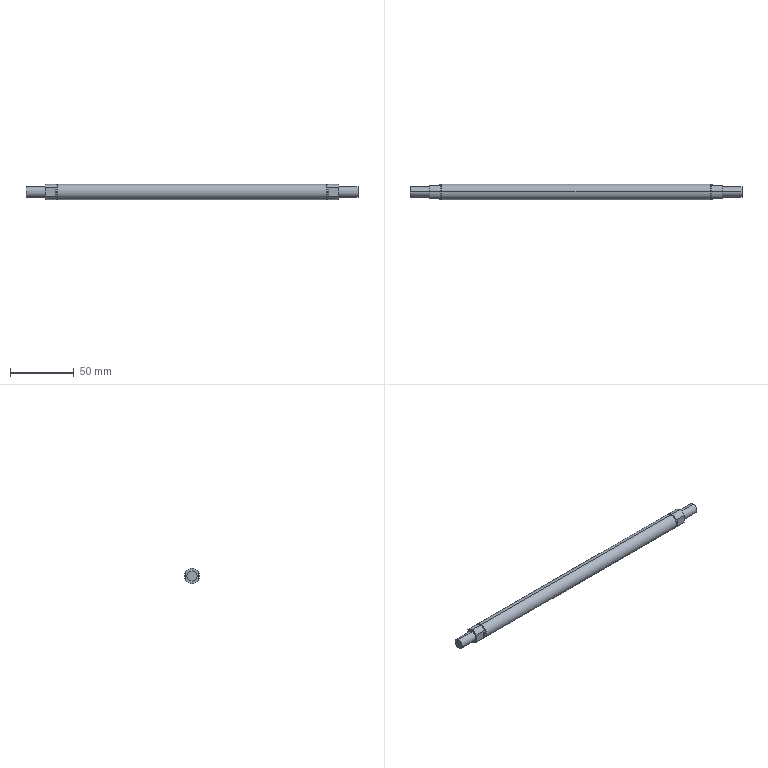Component | SolidWorks | GuideWheelAssembly3-1_RollerAxis2-1 | 1 solid | 30 faces | box 260 x 12 x 12 mm | volume 27307 mm3 | plane 16 | cylinder 14 | commonest cylinder face diameters 12 x6 10 x4 8 x4
build123d program:
from build123d import *

# Parameters (mm, degrees)
SKETCH1_R           = 6
BOSS_EXTRUDE1_DEPTH = 115
SKETCH3_R           = 4
BOSS_EXTRUDE2_DEPTH = 15
CUT_EXTRUDE7_START  = -8
CUT_EXTRUDE7_DEPTH  = 8
SKETCH20_W          = 1
SKETCH20_H          = 1


with BuildPart() as part:
    # Sketch1 → Boss-Extrude1 (new body)
    with BuildSketch(Plane(origin=(0, 0, 0), x_dir=(1, 0, 0), z_dir=(0, 1, 0))):
        with Locations(Location((0, 0, 0), (0, 0, 270))):
            Circle(SKETCH1_R)
    extrude(amount=BOSS_EXTRUDE1_DEPTH)

    # Sketch3 → Boss-Extrude2 (add)
    with BuildSketch(Plane(origin=(0, 115, 0), x_dir=(1, 0, 0), z_dir=(0, 1, 0))):
        with Locations(Location((0, 0, 0), (0, 0, 270))):
            Circle(SKETCH3_R)
    extrude(amount=BOSS_EXTRUDE2_DEPTH)

    # Sketch17 → Cut-Extrude7 (cut)
    with BuildSketch(Plane(origin=(0, 115, 0), x_dir=(1, 0, 0), z_dir=(0, 1, 0)).offset(CUT_EXTRUDE7_START)):
        with BuildLine():
            Line((-5, 3.317), (-5, -3.317))
            ThreePointArc((-5, -3.317), (-6, 0), (-5, 3.317))
        make_face()
        with BuildLine():
            Line((5, 3.317), (5, -3.317))
            ThreePointArc((5, -3.317), (6, 0), (5, 3.317))
        make_face()
    extrude(amount=CUT_EXTRUDE7_DEPTH, mode=Mode.SUBTRACT)

    # Sketch20 → Cut-Revolve1 (revolve, cut)
    with BuildSketch(Plane(origin=(0, 0, 0), x_dir=(0, 0, -1), z_dir=(1, 0, 0)), mode=Mode.PRIVATE) as cut_revolve1_sk:
        with Locations((5.5, 105.5)):
            Rectangle(SKETCH20_W, SKETCH20_H)
    revolve(cut_revolve1_sk.sketch.rotate(Axis((0, 130, 0), (0, -1, 0)), 180), axis=Axis((0, 130, 0), (0, -1, 0)), mode=Mode.SUBTRACT)

    # Mirror1: part across plane


with BuildPart() as part_1:
    add(part.part)
    add(part.part.mirror(Plane.ZX))


solid = part_1.part

# Placed as in the assembly
solid = solid.moved(Location((-394.97, -235, 30), (0, 0, 90)))
STEP:
#1=COLOUR_RGB('',0.7922,0.8196,0.9333);
#2=FILL_AREA_STYLE_COLOUR('',#1);
#3=FILL_AREA_STYLE('',(#2));
#4=SURFACE_STYLE_FILL_AREA(#3);
#5=SURFACE_SIDE_STYLE('',(#4));
#6=SURFACE_STYLE_USAGE(.BOTH.,#5);
#7=PRESENTATION_STYLE_ASSIGNMENT((#6));
#8=CARTESIAN_POINT('',(-11.416,-9.252,1.378));
#9=VERTEX_POINT('',#8);
#10=CARTESIAN_POINT('',(-11.416,-9.252,0.9843));
#11=VERTEX_POINT('',#10);
#12=CARTESIAN_POINT('',(-11.416,-9.252,1.181));
#13=DIRECTION('',(-1.,-0.,-0.));
#14=DIRECTION('',(0.,0.,-1.));
#15=AXIS2_PLACEMENT_3D('',#12,#13,#14);
#16=CIRCLE('',#15,0.1969);
#17=EDGE_CURVE('',#9,#11,#16,.T.);
#18=ORIENTED_EDGE('',*,*,#17,.F.);
#19=CARTESIAN_POINT('',(-11.377,-9.252,1.378));
#20=VERTEX_POINT('',#19);
#21=CARTESIAN_POINT('',(-10.432,-9.252,1.378));
#22=DIRECTION('',(1.,0.,0.));
#23=VECTOR('',#22,39.37);
#24=LINE('',#21,#23);
#25=EDGE_CURVE('',#9,#20,#24,.T.);
#26=ORIENTED_EDGE('',*,*,#25,.T.);
#27=CARTESIAN_POINT('',(-11.377,-9.252,0.9843));
#28=VERTEX_POINT('',#27);
#29=CARTESIAN_POINT('',(-11.377,-9.252,1.181));
#30=DIRECTION('',(-1.,-0.,-0.));
#31=DIRECTION('',(0.,0.,-1.));
#32=AXIS2_PLACEMENT_3D('',#29,#30,#31);
#33=CIRCLE('',#32,0.1969);
#34=EDGE_CURVE('',#20,#28,#33,.T.);
#35=ORIENTED_EDGE('',*,*,#34,.T.);
#36=CARTESIAN_POINT('',(-10.432,-9.252,0.9843));
#37=DIRECTION('',(1.,0.,0.));
#38=VECTOR('',#37,39.37);
#39=LINE('',#36,#38);
#40=EDGE_CURVE('',#11,#28,#39,.T.);
#41=ORIENTED_EDGE('',*,*,#40,.F.);
#42=EDGE_LOOP('',(#18,#26,#35,#41));
#43=FACE_OUTER_BOUND('',#42,.T.);
#44=CARTESIAN_POINT('',(-10.432,-9.252,1.181));
#45=DIRECTION('',(1.,0.,0.));
#46=DIRECTION('',(0.,0.,-1.));
#47=AXIS2_PLACEMENT_3D('',#44,#45,#46);
#48=CYLINDRICAL_SURFACE('',#47,0.1969);
#49=ADVANCED_FACE('',(#43),#48,.T.);
#50=CARTESIAN_POINT('',(-10.432,-9.252,1.339));
#51=VERTEX_POINT('',#50);
#52=CARTESIAN_POINT('',(-10.432,-9.252,1.024));
#53=VERTEX_POINT('',#52);
#54=CARTESIAN_POINT('',(-10.432,-9.252,1.181));
#55=DIRECTION('',(-1.,-0.,-0.));
#56=DIRECTION('',(0.,0.,-1.));
#57=AXIS2_PLACEMENT_3D('',#54,#55,#56);
#58=CIRCLE('',#57,0.1575);
#59=EDGE_CURVE('',#51,#53,#58,.T.);
#60=ORIENTED_EDGE('',*,*,#59,.T.);
#61=CARTESIAN_POINT('',(-11.022,-9.252,1.024));
#62=VERTEX_POINT('',#61);
#63=CARTESIAN_POINT('',(-10.432,-9.252,1.024));
#64=DIRECTION('',(-1.,-0.,-0.));
#65=VECTOR('',#64,39.37);
#66=LINE('',#63,#65);
#67=EDGE_CURVE('',#53,#62,#66,.T.);
#68=ORIENTED_EDGE('',*,*,#67,.T.);
#69=CARTESIAN_POINT('',(-11.022,-9.252,1.339));
#70=VERTEX_POINT('',#69);
#71=CARTESIAN_POINT('',(-11.022,-9.252,1.181));
#72=DIRECTION('',(-1.,-0.,-0.));
#73=DIRECTION('',(0.,0.,-1.));
#74=AXIS2_PLACEMENT_3D('',#71,#72,#73);
#75=CIRCLE('',#74,0.1575);
#76=EDGE_CURVE('',#70,#62,#75,.T.);
#77=ORIENTED_EDGE('',*,*,#76,.F.);
#78=CARTESIAN_POINT('',(-10.432,-9.252,1.339));
#79=DIRECTION('',(-1.,-0.,-0.));
#80=VECTOR('',#79,39.37);
#81=LINE('',#78,#80);
#82=EDGE_CURVE('',#51,#70,#81,.T.);
#83=ORIENTED_EDGE('',*,*,#82,.F.);
#84=EDGE_LOOP('',(#60,#68,#77,#83));
#85=FACE_OUTER_BOUND('',#84,.T.);
#86=CARTESIAN_POINT('',(-10.432,-9.252,1.181));
#87=DIRECTION('',(-1.,-0.,-0.));
#88=DIRECTION('',(0.,0.,1.));
#89=AXIS2_PLACEMENT_3D('',#86,#87,#88);
#90=CYLINDRICAL_SURFACE('',#89,0.1575);
#91=ADVANCED_FACE('',(#85),#90,.T.);
#92=CARTESIAN_POINT('',(-11.022,-9.055,1.051));
#93=VERTEX_POINT('',#92);
#94=CARTESIAN_POINT('',(-11.022,-9.252,0.9449));
#95=VERTEX_POINT('',#94);
#96=CARTESIAN_POINT('',(-11.022,-9.252,1.181));
#97=DIRECTION('',(-1.,-0.,-0.));
#98=DIRECTION('',(0.,0.,-1.));
#99=AXIS2_PLACEMENT_3D('',#96,#97,#98);
#100=CIRCLE('',#99,0.2362);
#101=EDGE_CURVE('',#93,#95,#100,.T.);
#102=ORIENTED_EDGE('',*,*,#101,.T.);
#103=CARTESIAN_POINT('',(-11.377,-9.252,0.9449));
#104=VERTEX_POINT('',#103);
#105=CARTESIAN_POINT('',(-11.022,-9.252,0.9449));
#106=DIRECTION('',(-1.,-0.,-0.));
#107=VECTOR('',#106,39.37);
#108=LINE('',#105,#107);
#109=EDGE_CURVE('',#95,#104,#108,.T.);
#110=ORIENTED_EDGE('',*,*,#109,.T.);
#111=CARTESIAN_POINT('',(-11.377,-9.252,1.417));
#112=VERTEX_POINT('',#111);
#113=CARTESIAN_POINT('',(-11.377,-9.252,1.181));
#114=DIRECTION('',(-1.,-0.,-0.));
#115=DIRECTION('',(0.,0.,-1.));
#116=AXIS2_PLACEMENT_3D('',#113,#114,#115);
#117=CIRCLE('',#116,0.2362);
#118=EDGE_CURVE('',#112,#104,#117,.T.);
#119=ORIENTED_EDGE('',*,*,#118,.F.);
#120=CARTESIAN_POINT('',(-11.022,-9.252,1.417));
#121=VERTEX_POINT('',#120);
#122=CARTESIAN_POINT('',(-11.022,-9.252,1.417));
#123=DIRECTION('',(-1.,-0.,-0.));
#124=VECTOR('',#123,39.37);
#125=LINE('',#122,#124);
#126=EDGE_CURVE('',#121,#112,#125,.T.);
#127=ORIENTED_EDGE('',*,*,#126,.F.);
#128=CARTESIAN_POINT('',(-11.022,-9.055,1.312));
#129=VERTEX_POINT('',#128);
#130=CARTESIAN_POINT('',(-11.022,-9.252,1.181));
#131=DIRECTION('',(-1.,-0.,-0.));
#132=DIRECTION('',(0.,0.,-1.));
#133=AXIS2_PLACEMENT_3D('',#130,#131,#132);
#134=CIRCLE('',#133,0.2362);
#135=EDGE_CURVE('',#121,#129,#134,.T.);
#136=ORIENTED_EDGE('',*,*,#135,.T.);
#137=CARTESIAN_POINT('',(-11.337,-9.055,1.312));
#138=VERTEX_POINT('',#137);
#139=CARTESIAN_POINT('',(-11.337,-9.055,1.312));
#140=DIRECTION('',(1.,0.,0.));
#141=VECTOR('',#140,39.37);
#142=LINE('',#139,#141);
#143=EDGE_CURVE('',#138,#129,#142,.T.);
#144=ORIENTED_EDGE('',*,*,#143,.F.);
#145=CARTESIAN_POINT('',(-11.337,-9.055,1.051));
#146=VERTEX_POINT('',#145);
#147=CARTESIAN_POINT('',(-11.337,-9.252,1.181));
#148=DIRECTION('',(-1.,-0.,-0.));
#149=DIRECTION('',(0.,0.,-1.));
#150=AXIS2_PLACEMENT_3D('',#147,#148,#149);
#151=CIRCLE('',#150,0.2362);
#152=EDGE_CURVE('',#138,#146,#151,.T.);
#153=ORIENTED_EDGE('',*,*,#152,.T.);
#154=CARTESIAN_POINT('',(-11.337,-9.055,1.051));
#155=DIRECTION('',(1.,0.,0.));
#156=VECTOR('',#155,39.37);
#157=LINE('',#154,#156);
#158=EDGE_CURVE('',#146,#93,#157,.T.);
#159=ORIENTED_EDGE('',*,*,#158,.T.);
#160=EDGE_LOOP('',(#102,#110,#119,#127,#136,#144,#153,#159));
#161=FACE_OUTER_BOUND('',#160,.T.);
#162=CARTESIAN_POINT('',(-11.022,-9.252,1.181));
#163=DIRECTION('',(-1.,-0.,-0.));
#164=DIRECTION('',(0.,0.,1.));
#165=AXIS2_PLACEMENT_3D('',#162,#163,#164);
#166=CYLINDRICAL_SURFACE('',#165,0.2362);
#167=ADVANCED_FACE('',(#161),#166,.T.);
#168=CARTESIAN_POINT('',(-19.684,-9.252,0.9449));
#169=VERTEX_POINT('',#168);
#170=CARTESIAN_POINT('',(-19.684,-9.252,1.417));
#171=VERTEX_POINT('',#170);
#172=CARTESIAN_POINT('',(-19.684,-9.252,1.181));
#173=DIRECTION('',(-1.,-0.,-0.));
#174=DIRECTION('',(0.,0.,-1.));
#175=AXIS2_PLACEMENT_3D('',#172,#173,#174);
#176=CIRCLE('',#175,0.2362);
#177=EDGE_CURVE('',#169,#171,#176,.T.);
#178=ORIENTED_EDGE('',*,*,#177,.F.);
#179=CARTESIAN_POINT('',(-11.416,-9.252,0.9449));
#180=VERTEX_POINT('',#179);
#181=CARTESIAN_POINT('',(-20.078,-9.252,0.9449));
#182=DIRECTION('',(1.,0.,0.));
#183=VECTOR('',#182,39.37);
#184=LINE('',#181,#183);
#185=EDGE_CURVE('',#169,#180,#184,.T.);
#186=ORIENTED_EDGE('',*,*,#185,.T.);
#187=CARTESIAN_POINT('',(-11.416,-9.252,1.417));
#188=VERTEX_POINT('',#187);
#189=CARTESIAN_POINT('',(-11.416,-9.252,1.181));
#190=DIRECTION('',(-1.,-0.,-0.));
#191=DIRECTION('',(0.,0.,-1.));
#192=AXIS2_PLACEMENT_3D('',#189,#190,#191);
#193=CIRCLE('',#192,0.2362);
#194=EDGE_CURVE('',#180,#188,#193,.T.);
#195=ORIENTED_EDGE('',*,*,#194,.T.);
#196=CARTESIAN_POINT('',(-20.078,-9.252,1.417));
#197=DIRECTION('',(1.,0.,0.));
#198=VECTOR('',#197,39.37);
#199=LINE('',#196,#198);
#200=EDGE_CURVE('',#171,#188,#199,.T.);
#201=ORIENTED_EDGE('',*,*,#200,.F.);
#202=EDGE_LOOP('',(#178,#186,#195,#201));
#203=FACE_OUTER_BOUND('',#202,.T.);
#204=CARTESIAN_POINT('',(-20.078,-9.252,1.181));
#205=DIRECTION('',(1.,0.,0.));
#206=DIRECTION('',(0.,0.,1.));
#207=AXIS2_PLACEMENT_3D('',#204,#205,#206);
#208=CYLINDRICAL_SURFACE('',#207,0.2362);
#209=ADVANCED_FACE('',(#203),#208,.T.);
#210=CARTESIAN_POINT('',(-19.684,-9.252,0.9843));
#211=VERTEX_POINT('',#210);
#212=CARTESIAN_POINT('',(-19.684,-9.252,1.378));
#213=VERTEX_POINT('',#212);
#214=CARTESIAN_POINT('',(-19.684,-9.252,1.181));
#215=DIRECTION('',(-1.,-0.,-0.));
#216=DIRECTION('',(0.,0.,-1.));
#217=AXIS2_PLACEMENT_3D('',#214,#215,#216);
#218=CIRCLE('',#217,0.1969);
#219=EDGE_CURVE('',#211,#213,#218,.T.);
#220=ORIENTED_EDGE('',*,*,#219,.T.);
#221=CARTESIAN_POINT('',(-19.723,-9.252,1.378));
#222=VERTEX_POINT('',#221);
#223=CARTESIAN_POINT('',(-20.668,-9.252,1.378));
#224=DIRECTION('',(-1.,-0.,-0.));
#225=VECTOR('',#224,39.37);
#226=LINE('',#223,#225);
#227=EDGE_CURVE('',#213,#222,#226,.T.);
#228=ORIENTED_EDGE('',*,*,#227,.T.);
#229=CARTESIAN_POINT('',(-19.723,-9.252,0.9843));
#230=VERTEX_POINT('',#229);
#231=CARTESIAN_POINT('',(-19.723,-9.252,1.181));
#232=DIRECTION('',(-1.,-0.,-0.));
#233=DIRECTION('',(0.,0.,-1.));
#234=AXIS2_PLACEMENT_3D('',#231,#232,#233);
#235=CIRCLE('',#234,0.1969);
#236=EDGE_CURVE('',#230,#222,#235,.T.);
#237=ORIENTED_EDGE('',*,*,#236,.F.);
#238=CARTESIAN_POINT('',(-20.668,-9.252,0.9843));
#239=DIRECTION('',(-1.,-0.,-0.));
#240=VECTOR('',#239,39.37);
#241=LINE('',#238,#240);
#242=EDGE_CURVE('',#211,#230,#241,.T.);
#243=ORIENTED_EDGE('',*,*,#242,.F.);
#244=EDGE_LOOP('',(#220,#228,#237,#243));
#245=FACE_OUTER_BOUND('',#244,.T.);
#246=CARTESIAN_POINT('',(-20.668,-9.252,1.181));
#247=DIRECTION('',(-1.,-0.,-0.));
#248=DIRECTION('',(0.,0.,-1.));
#249=AXIS2_PLACEMENT_3D('',#246,#247,#248);
#250=CYLINDRICAL_SURFACE('',#249,0.1969);
#251=ADVANCED_FACE('',(#245),#250,.T.);
#252=CARTESIAN_POINT('',(-20.668,-9.252,1.024));
#253=VERTEX_POINT('',#252);
#254=CARTESIAN_POINT('',(-20.668,-9.252,1.339));
#255=VERTEX_POINT('',#254);
#256=CARTESIAN_POINT('',(-20.668,-9.252,1.181));
#257=DIRECTION('',(-1.,-0.,-0.));
#258=DIRECTION('',(0.,0.,-1.));
#259=AXIS2_PLACEMENT_3D('',#256,#257,#258);
#260=CIRCLE('',#259,0.1575);
#261=EDGE_CURVE('',#253,#255,#260,.T.);
#262=ORIENTED_EDGE('',*,*,#261,.F.);
#263=CARTESIAN_POINT('',(-20.078,-9.252,1.024));
#264=VERTEX_POINT('',#263);
#265=CARTESIAN_POINT('',(-20.668,-9.252,1.024));
#266=DIRECTION('',(1.,0.,0.));
#267=VECTOR('',#266,39.37);
#268=LINE('',#265,#267);
#269=EDGE_CURVE('',#253,#264,#268,.T.);
#270=ORIENTED_EDGE('',*,*,#269,.T.);
#271=CARTESIAN_POINT('',(-20.078,-9.252,1.339));
#272=VERTEX_POINT('',#271);
#273=CARTESIAN_POINT('',(-20.078,-9.252,1.181));
#274=DIRECTION('',(-1.,-0.,-0.));
#275=DIRECTION('',(0.,0.,-1.));
#276=AXIS2_PLACEMENT_3D('',#273,#274,#275);
#277=CIRCLE('',#276,0.1575);
#278=EDGE_CURVE('',#264,#272,#277,.T.);
#279=ORIENTED_EDGE('',*,*,#278,.T.);
#280=CARTESIAN_POINT('',(-20.668,-9.252,1.339));
#281=DIRECTION('',(1.,0.,0.));
#282=VECTOR('',#281,39.37);
#283=LINE('',#280,#282);
#284=EDGE_CURVE('',#255,#272,#283,.T.);
#285=ORIENTED_EDGE('',*,*,#284,.F.);
#286=EDGE_LOOP('',(#262,#270,#279,#285));
#287=FACE_OUTER_BOUND('',#286,.T.);
#288=CARTESIAN_POINT('',(-20.668,-9.252,1.181));
#289=DIRECTION('',(1.,0.,0.));
#290=DIRECTION('',(0.,0.,1.));
#291=AXIS2_PLACEMENT_3D('',#288,#289,#290);
#292=CYLINDRICAL_SURFACE('',#291,0.1575);
#293=ADVANCED_FACE('',(#287),#292,.T.);
#294=CARTESIAN_POINT('',(-20.078,-9.252,0.9449));
#295=VERTEX_POINT('',#294);
#296=CARTESIAN_POINT('',(-20.078,-9.449,1.051));
#297=VERTEX_POINT('',#296);
#298=CARTESIAN_POINT('',(-20.078,-9.252,1.181));
#299=DIRECTION('',(-1.,-0.,-0.));
#300=DIRECTION('',(0.,0.,-1.));
#301=AXIS2_PLACEMENT_3D('',#298,#299,#300);
#302=CIRCLE('',#301,0.2362);
#303=EDGE_CURVE('',#295,#297,#302,.T.);
#304=ORIENTED_EDGE('',*,*,#303,.F.);
#305=CARTESIAN_POINT('',(-19.723,-9.252,0.9449));
#306=VERTEX_POINT('',#305);
#307=CARTESIAN_POINT('',(-20.078,-9.252,0.9449));
#308=DIRECTION('',(1.,0.,0.));
#309=VECTOR('',#308,39.37);
#310=LINE('',#307,#309);
#311=EDGE_CURVE('',#295,#306,#310,.T.);
#312=ORIENTED_EDGE('',*,*,#311,.T.);
#313=CARTESIAN_POINT('',(-19.723,-9.252,1.417));
#314=VERTEX_POINT('',#313);
#315=CARTESIAN_POINT('',(-19.723,-9.252,1.181));
#316=DIRECTION('',(-1.,-0.,-0.));
#317=DIRECTION('',(0.,0.,-1.));
#318=AXIS2_PLACEMENT_3D('',#315,#316,#317);
#319=CIRCLE('',#318,0.2362);
#320=EDGE_CURVE('',#306,#314,#319,.T.);
#321=ORIENTED_EDGE('',*,*,#320,.T.);
#322=CARTESIAN_POINT('',(-20.078,-9.252,1.417));
#323=VERTEX_POINT('',#322);
#324=CARTESIAN_POINT('',(-20.078,-9.252,1.417));
#325=DIRECTION('',(1.,0.,0.));
#326=VECTOR('',#325,39.37);
#327=LINE('',#324,#326);
#328=EDGE_CURVE('',#323,#314,#327,.T.);
#329=ORIENTED_EDGE('',*,*,#328,.F.);
#330=CARTESIAN_POINT('',(-20.078,-9.449,1.312));
#331=VERTEX_POINT('',#330);
#332=CARTESIAN_POINT('',(-20.078,-9.252,1.181));
#333=DIRECTION('',(-1.,-0.,-0.));
#334=DIRECTION('',(0.,0.,-1.));
#335=AXIS2_PLACEMENT_3D('',#332,#333,#334);
#336=CIRCLE('',#335,0.2362);
#337=EDGE_CURVE('',#331,#323,#336,.T.);
#338=ORIENTED_EDGE('',*,*,#337,.F.);
#339=CARTESIAN_POINT('',(-19.763,-9.449,1.312));
#340=VERTEX_POINT('',#339);
#341=CARTESIAN_POINT('',(-19.763,-9.449,1.312));
#342=DIRECTION('',(-1.,-0.,-0.));
#343=VECTOR('',#342,39.37);
#344=LINE('',#341,#343);
#345=EDGE_CURVE('',#340,#331,#344,.T.);
#346=ORIENTED_EDGE('',*,*,#345,.F.);
#347=CARTESIAN_POINT('',(-19.763,-9.449,1.051));
#348=VERTEX_POINT('',#347);
#349=CARTESIAN_POINT('',(-19.763,-9.252,1.181));
#350=DIRECTION('',(-1.,-0.,-0.));
#351=DIRECTION('',(0.,0.,-1.));
#352=AXIS2_PLACEMENT_3D('',#349,#350,#351);
#353=CIRCLE('',#352,0.2362);
#354=EDGE_CURVE('',#348,#340,#353,.T.);
#355=ORIENTED_EDGE('',*,*,#354,.F.);
#356=CARTESIAN_POINT('',(-19.763,-9.449,1.051));
#357=DIRECTION('',(-1.,-0.,-0.));
#358=VECTOR('',#357,39.37);
#359=LINE('',#356,#358);
#360=EDGE_CURVE('',#348,#297,#359,.T.);
#361=ORIENTED_EDGE('',*,*,#360,.T.);
#362=EDGE_LOOP('',(#304,#312,#321,#329,#338,#346,#355,#361));
#363=FACE_OUTER_BOUND('',#362,.T.);
#364=CARTESIAN_POINT('',(-20.078,-9.252,1.181));
#365=DIRECTION('',(1.,0.,0.));
#366=DIRECTION('',(0.,0.,1.));
#367=AXIS2_PLACEMENT_3D('',#364,#365,#366);
#368=CYLINDRICAL_SURFACE('',#367,0.2362);
#369=ADVANCED_FACE('',(#363),#368,.T.);
#370=ORIENTED_EDGE('',*,*,#311,.F.);
#371=CARTESIAN_POINT('',(-20.078,-9.055,1.051));
#372=VERTEX_POINT('',#371);
#373=CARTESIAN_POINT('',(-20.078,-9.252,1.181));
#374=DIRECTION('',(-1.,-0.,-0.));
#375=DIRECTION('',(0.,0.,-1.));
#376=AXIS2_PLACEMENT_3D('',#373,#374,#375);
#377=CIRCLE('',#376,0.2362);
#378=EDGE_CURVE('',#372,#295,#377,.T.);
#379=ORIENTED_EDGE('',*,*,#378,.F.);
#380=CARTESIAN_POINT('',(-19.763,-9.055,1.051));
#381=VERTEX_POINT('',#380);
#382=CARTESIAN_POINT('',(-19.763,-9.055,1.051));
#383=DIRECTION('',(-1.,-0.,-0.));
#384=VECTOR('',#383,39.37);
#385=LINE('',#382,#384);
#386=EDGE_CURVE('',#381,#372,#385,.T.);
#387=ORIENTED_EDGE('',*,*,#386,.F.);
#388=CARTESIAN_POINT('',(-19.763,-9.055,1.312));
#389=VERTEX_POINT('',#388);
#390=CARTESIAN_POINT('',(-19.763,-9.252,1.181));
#391=DIRECTION('',(-1.,-0.,-0.));
#392=DIRECTION('',(0.,0.,-1.));
#393=AXIS2_PLACEMENT_3D('',#390,#391,#392);
#394=CIRCLE('',#393,0.2362);
#395=EDGE_CURVE('',#389,#381,#394,.T.);
#396=ORIENTED_EDGE('',*,*,#395,.F.);
#397=CARTESIAN_POINT('',(-20.078,-9.055,1.312));
#398=VERTEX_POINT('',#397);
#399=CARTESIAN_POINT('',(-19.763,-9.055,1.312));
#400=DIRECTION('',(-1.,-0.,-0.));
#401=VECTOR('',#400,39.37);
#402=LINE('',#399,#401);
#403=EDGE_CURVE('',#389,#398,#402,.T.);
#404=ORIENTED_EDGE('',*,*,#403,.T.);
#405=CARTESIAN_POINT('',(-20.078,-9.252,1.181));
#406=DIRECTION('',(-1.,-0.,-0.));
#407=DIRECTION('',(0.,0.,-1.));
#408=AXIS2_PLACEMENT_3D('',#405,#406,#407);
#409=CIRCLE('',#408,0.2362);
#410=EDGE_CURVE('',#323,#398,#409,.T.);
#411=ORIENTED_EDGE('',*,*,#410,.F.);
#412=ORIENTED_EDGE('',*,*,#328,.T.);
#413=CARTESIAN_POINT('',(-19.723,-9.252,1.181));
#414=DIRECTION('',(-1.,-0.,-0.));
#415=DIRECTION('',(0.,0.,-1.));
#416=AXIS2_PLACEMENT_3D('',#413,#414,#415);
#417=CIRCLE('',#416,0.2362);
#418=EDGE_CURVE('',#314,#306,#417,.T.);
#419=ORIENTED_EDGE('',*,*,#418,.T.);
#420=EDGE_LOOP('',(#370,#379,#387,#396,#404,#411,#412,#419));
#421=FACE_OUTER_BOUND('',#420,.T.);
#422=CARTESIAN_POINT('',(-20.078,-9.252,1.181));
#423=DIRECTION('',(1.,0.,0.));
#424=DIRECTION('',(0.,0.,1.));
#425=AXIS2_PLACEMENT_3D('',#422,#423,#424);
#426=CYLINDRICAL_SURFACE('',#425,0.2362);
#427=ADVANCED_FACE('',(#421),#426,.T.);
#428=CARTESIAN_POINT('',(-20.078,-9.055,1.312));
#429=DIRECTION('',(-0.,0.,1.));
#430=VECTOR('',#429,39.37);
#431=LINE('',#428,#430);
#432=EDGE_CURVE('',#372,#398,#431,.T.);
#433=ORIENTED_EDGE('',*,*,#432,.F.);
#434=ORIENTED_EDGE('',*,*,#378,.T.);
#435=ORIENTED_EDGE('',*,*,#303,.T.);
#436=CARTESIAN_POINT('',(-20.078,-9.449,1.312));
#437=DIRECTION('',(0.,-0.,-1.));
#438=VECTOR('',#437,39.37);
#439=LINE('',#436,#438);
#440=EDGE_CURVE('',#331,#297,#439,.T.);
#441=ORIENTED_EDGE('',*,*,#440,.F.);
#442=ORIENTED_EDGE('',*,*,#337,.T.);
#443=ORIENTED_EDGE('',*,*,#410,.T.);
#444=EDGE_LOOP('',(#433,#434,#435,#441,#442,#443));
#445=FACE_OUTER_BOUND('',#444,.T.);
#446=CARTESIAN_POINT('',(-20.078,-9.252,1.181));
#447=DIRECTION('',(-1.,-0.,-0.));
#448=DIRECTION('',(0.,0.,-1.));
#449=AXIS2_PLACEMENT_3D('',#446,#447,#448);
#450=CIRCLE('',#449,0.1575);
#451=EDGE_CURVE('',#272,#264,#450,.T.);
#452=ORIENTED_EDGE('',*,*,#451,.F.);
#453=ORIENTED_EDGE('',*,*,#278,.F.);
#454=EDGE_LOOP('',(#452,#453));
#455=FACE_BOUND('',#454,.T.);
#456=CARTESIAN_POINT('',(-20.078,-9.252,1.181));
#457=DIRECTION('',(-1.,-0.,-0.));
#458=DIRECTION('',(0.,-0.,-1.));
#459=AXIS2_PLACEMENT_3D('',#456,#457,#458);
#460=PLANE('',#459);
#461=ADVANCED_FACE('',(#445,#455),#460,.T.);
#462=ORIENTED_EDGE('',*,*,#269,.F.);
#463=CARTESIAN_POINT('',(-20.668,-9.252,1.181));
#464=DIRECTION('',(-1.,-0.,-0.));
#465=DIRECTION('',(0.,0.,-1.));
#466=AXIS2_PLACEMENT_3D('',#463,#464,#465);
#467=CIRCLE('',#466,0.1575);
#468=EDGE_CURVE('',#255,#253,#467,.T.);
#469=ORIENTED_EDGE('',*,*,#468,.F.);
#470=ORIENTED_EDGE('',*,*,#284,.T.);
#471=ORIENTED_EDGE('',*,*,#451,.T.);
#472=EDGE_LOOP('',(#462,#469,#470,#471));
#473=FACE_OUTER_BOUND('',#472,.T.);
#474=CARTESIAN_POINT('',(-20.668,-9.252,1.181));
#475=DIRECTION('',(1.,0.,0.));
#476=DIRECTION('',(0.,0.,1.));
#477=AXIS2_PLACEMENT_3D('',#474,#475,#476);
#478=CYLINDRICAL_SURFACE('',#477,0.1575);
#479=ADVANCED_FACE('',(#473),#478,.T.);
#480=ORIENTED_EDGE('',*,*,#468,.T.);
#481=ORIENTED_EDGE('',*,*,#261,.T.);
#482=EDGE_LOOP('',(#480,#481));
#483=FACE_OUTER_BOUND('',#482,.T.);
#484=CARTESIAN_POINT('',(-20.668,-9.252,1.181));
#485=DIRECTION('',(-1.,-0.,-0.));
#486=DIRECTION('',(0.,-0.,-1.));
#487=AXIS2_PLACEMENT_3D('',#484,#485,#486);
#488=PLANE('',#487);
#489=ADVANCED_FACE('',(#483),#488,.T.);
#490=ORIENTED_EDGE('',*,*,#440,.T.);
#491=ORIENTED_EDGE('',*,*,#360,.F.);
#492=CARTESIAN_POINT('',(-19.763,-9.449,1.312));
#493=DIRECTION('',(0.,-0.,-1.));
#494=VECTOR('',#493,39.37);
#495=LINE('',#492,#494);
#496=EDGE_CURVE('',#340,#348,#495,.T.);
#497=ORIENTED_EDGE('',*,*,#496,.F.);
#498=ORIENTED_EDGE('',*,*,#345,.T.);
#499=EDGE_LOOP('',(#490,#491,#497,#498));
#500=FACE_OUTER_BOUND('',#499,.T.);
#501=CARTESIAN_POINT('',(-19.763,-9.449,1.312));
#502=DIRECTION('',(-0.,1.,-0.));
#503=DIRECTION('',(0.,-0.,-1.));
#504=AXIS2_PLACEMENT_3D('',#501,#502,#503);
#505=PLANE('',#504);
#506=ADVANCED_FACE('',(#500),#505,.F.);
#507=ORIENTED_EDGE('',*,*,#354,.T.);
#508=ORIENTED_EDGE('',*,*,#496,.T.);
#509=EDGE_LOOP('',(#507,#508));
#510=FACE_OUTER_BOUND('',#509,.T.);
#511=CARTESIAN_POINT('',(-19.763,-9.252,1.181));
#512=DIRECTION('',(-1.,-0.,-0.));
#513=DIRECTION('',(0.,-0.,-1.));
#514=AXIS2_PLACEMENT_3D('',#511,#512,#513);
#515=PLANE('',#514);
#516=ADVANCED_FACE('',(#510),#515,.T.);
#517=ORIENTED_EDGE('',*,*,#432,.T.);
#518=ORIENTED_EDGE('',*,*,#403,.F.);
#519=CARTESIAN_POINT('',(-19.763,-9.055,1.312));
#520=DIRECTION('',(-0.,0.,1.));
#521=VECTOR('',#520,39.37);
#522=LINE('',#519,#521);
#523=EDGE_CURVE('',#381,#389,#522,.T.);
#524=ORIENTED_EDGE('',*,*,#523,.F.);
#525=ORIENTED_EDGE('',*,*,#386,.T.);
#526=EDGE_LOOP('',(#517,#518,#524,#525));
#527=FACE_OUTER_BOUND('',#526,.T.);
#528=CARTESIAN_POINT('',(-19.763,-9.055,1.312));
#529=DIRECTION('',(0.,-1.,0.));
#530=DIRECTION('',(-0.,0.,1.));
#531=AXIS2_PLACEMENT_3D('',#528,#529,#530);
#532=PLANE('',#531);
#533=ADVANCED_FACE('',(#527),#532,.F.);
#534=ORIENTED_EDGE('',*,*,#395,.T.);
#535=ORIENTED_EDGE('',*,*,#523,.T.);
#536=EDGE_LOOP('',(#534,#535));
#537=FACE_OUTER_BOUND('',#536,.T.);
#538=CARTESIAN_POINT('',(-19.763,-9.252,1.181));
#539=DIRECTION('',(-1.,-0.,-0.));
#540=DIRECTION('',(0.,-0.,-1.));
#541=AXIS2_PLACEMENT_3D('',#538,#539,#540);
#542=PLANE('',#541);
#543=ADVANCED_FACE('',(#537),#542,.T.);
#544=CARTESIAN_POINT('',(-19.684,-9.252,1.181));
#545=DIRECTION('',(-1.,-0.,-0.));
#546=DIRECTION('',(0.,0.,-1.));
#547=AXIS2_PLACEMENT_3D('',#544,#545,#546);
#548=CIRCLE('',#547,0.2362);
#549=EDGE_CURVE('',#171,#169,#548,.T.);
#550=ORIENTED_EDGE('',*,*,#549,.T.);
#551=ORIENTED_EDGE('',*,*,#177,.T.);
#552=EDGE_LOOP('',(#550,#551));
#553=FACE_OUTER_BOUND('',#552,.T.);
#554=ORIENTED_EDGE('',*,*,#219,.F.);
#555=CARTESIAN_POINT('',(-19.684,-9.252,1.181));
#556=DIRECTION('',(-1.,-0.,-0.));
#557=DIRECTION('',(0.,0.,-1.));
#558=AXIS2_PLACEMENT_3D('',#555,#556,#557);
#559=CIRCLE('',#558,0.1969);
#560=EDGE_CURVE('',#213,#211,#559,.T.);
#561=ORIENTED_EDGE('',*,*,#560,.F.);
#562=EDGE_LOOP('',(#554,#561));
#563=FACE_BOUND('',#562,.T.);
#564=CARTESIAN_POINT('',(-19.684,-9.252,1.417));
#565=DIRECTION('',(-1.,-0.,-0.));
#566=DIRECTION('',(0.,-0.,-1.));
#567=AXIS2_PLACEMENT_3D('',#564,#565,#566);
#568=PLANE('',#567);
#569=ADVANCED_FACE('',(#553,#563),#568,.T.);
#570=ORIENTED_EDGE('',*,*,#227,.F.);
#571=ORIENTED_EDGE('',*,*,#560,.T.);
#572=ORIENTED_EDGE('',*,*,#242,.T.);
#573=CARTESIAN_POINT('',(-19.723,-9.252,1.181));
#574=DIRECTION('',(-1.,-0.,-0.));
#575=DIRECTION('',(0.,0.,-1.));
#576=AXIS2_PLACEMENT_3D('',#573,#574,#575);
#577=CIRCLE('',#576,0.1969);
#578=EDGE_CURVE('',#222,#230,#577,.T.);
#579=ORIENTED_EDGE('',*,*,#578,.F.);
#580=EDGE_LOOP('',(#570,#571,#572,#579));
#581=FACE_OUTER_BOUND('',#580,.T.);
#582=CARTESIAN_POINT('',(-20.668,-9.252,1.181));
#583=DIRECTION('',(-1.,-0.,-0.));
#584=DIRECTION('',(0.,0.,-1.));
#585=AXIS2_PLACEMENT_3D('',#582,#583,#584);
#586=CYLINDRICAL_SURFACE('',#585,0.1969);
#587=ADVANCED_FACE('',(#581),#586,.T.);
#588=ORIENTED_EDGE('',*,*,#236,.T.);
#589=ORIENTED_EDGE('',*,*,#578,.T.);
#590=EDGE_LOOP('',(#588,#589));
#591=FACE_BOUND('',#590,.T.);
#592=ORIENTED_EDGE('',*,*,#418,.F.);
#593=ORIENTED_EDGE('',*,*,#320,.F.);
#594=EDGE_LOOP('',(#592,#593));
#595=FACE_OUTER_BOUND('',#594,.T.);
#596=CARTESIAN_POINT('',(-19.723,-9.252,1.417));
#597=DIRECTION('',(1.,0.,0.));
#598=DIRECTION('',(-0.,0.,1.));
#599=AXIS2_PLACEMENT_3D('',#596,#597,#598);
#600=PLANE('',#599);
#601=ADVANCED_FACE('',(#591,#595),#600,.T.);
#602=ORIENTED_EDGE('',*,*,#185,.F.);
#603=ORIENTED_EDGE('',*,*,#549,.F.);
#604=ORIENTED_EDGE('',*,*,#200,.T.);
#605=CARTESIAN_POINT('',(-11.416,-9.252,1.181));
#606=DIRECTION('',(-1.,-0.,-0.));
#607=DIRECTION('',(0.,0.,-1.));
#608=AXIS2_PLACEMENT_3D('',#605,#606,#607);
#609=CIRCLE('',#608,0.2362);
#610=EDGE_CURVE('',#188,#180,#609,.T.);
#611=ORIENTED_EDGE('',*,*,#610,.T.);
#612=EDGE_LOOP('',(#602,#603,#604,#611));
#613=FACE_OUTER_BOUND('',#612,.T.);
#614=CARTESIAN_POINT('',(-20.078,-9.252,1.181));
#615=DIRECTION('',(1.,0.,0.));
#616=DIRECTION('',(0.,0.,1.));
#617=AXIS2_PLACEMENT_3D('',#614,#615,#616);
#618=CYLINDRICAL_SURFACE('',#617,0.2362);
#619=ADVANCED_FACE('',(#613),#618,.T.);
#620=ORIENTED_EDGE('',*,*,#109,.F.);
#621=CARTESIAN_POINT('',(-11.022,-9.449,1.051));
#622=VERTEX_POINT('',#621);
#623=CARTESIAN_POINT('',(-11.022,-9.252,1.181));
#624=DIRECTION('',(-1.,-0.,-0.));
#625=DIRECTION('',(0.,0.,-1.));
#626=AXIS2_PLACEMENT_3D('',#623,#624,#625);
#627=CIRCLE('',#626,0.2362);
#628=EDGE_CURVE('',#95,#622,#627,.T.);
#629=ORIENTED_EDGE('',*,*,#628,.T.);
#630=CARTESIAN_POINT('',(-11.337,-9.449,1.051));
#631=VERTEX_POINT('',#630);
#632=CARTESIAN_POINT('',(-11.337,-9.449,1.051));
#633=DIRECTION('',(1.,0.,0.));
#634=VECTOR('',#633,39.37);
#635=LINE('',#632,#634);
#636=EDGE_CURVE('',#631,#622,#635,.T.);
#637=ORIENTED_EDGE('',*,*,#636,.F.);
#638=CARTESIAN_POINT('',(-11.337,-9.449,1.312));
#639=VERTEX_POINT('',#638);
#640=CARTESIAN_POINT('',(-11.337,-9.252,1.181));
#641=DIRECTION('',(-1.,-0.,-0.));
#642=DIRECTION('',(0.,0.,-1.));
#643=AXIS2_PLACEMENT_3D('',#640,#641,#642);
#644=CIRCLE('',#643,0.2362);
#645=EDGE_CURVE('',#631,#639,#644,.T.);
#646=ORIENTED_EDGE('',*,*,#645,.T.);
#647=CARTESIAN_POINT('',(-11.022,-9.449,1.312));
#648=VERTEX_POINT('',#647);
#649=CARTESIAN_POINT('',(-11.337,-9.449,1.312));
#650=DIRECTION('',(1.,0.,0.));
#651=VECTOR('',#650,39.37);
#652=LINE('',#649,#651);
#653=EDGE_CURVE('',#639,#648,#652,.T.);
#654=ORIENTED_EDGE('',*,*,#653,.T.);
#655=CARTESIAN_POINT('',(-11.022,-9.252,1.181));
#656=DIRECTION('',(-1.,-0.,-0.));
#657=DIRECTION('',(0.,0.,-1.));
#658=AXIS2_PLACEMENT_3D('',#655,#656,#657);
#659=CIRCLE('',#658,0.2362);
#660=EDGE_CURVE('',#648,#121,#659,.T.);
#661=ORIENTED_EDGE('',*,*,#660,.T.);
#662=ORIENTED_EDGE('',*,*,#126,.T.);
#663=CARTESIAN_POINT('',(-11.377,-9.252,1.181));
#664=DIRECTION('',(-1.,-0.,-0.));
#665=DIRECTION('',(0.,0.,-1.));
#666=AXIS2_PLACEMENT_3D('',#663,#664,#665);
#667=CIRCLE('',#666,0.2362);
#668=EDGE_CURVE('',#104,#112,#667,.T.);
#669=ORIENTED_EDGE('',*,*,#668,.F.);
#670=EDGE_LOOP('',(#620,#629,#637,#646,#654,#661,#662,#669));
#671=FACE_OUTER_BOUND('',#670,.T.);
#672=CARTESIAN_POINT('',(-11.022,-9.252,1.181));
#673=DIRECTION('',(-1.,-0.,-0.));
#674=DIRECTION('',(0.,0.,1.));
#675=AXIS2_PLACEMENT_3D('',#672,#673,#674);
#676=CYLINDRICAL_SURFACE('',#675,0.2362);
#677=ADVANCED_FACE('',(#671),#676,.T.);
#678=CARTESIAN_POINT('',(-11.022,-9.055,1.312));
#679=DIRECTION('',(-0.,0.,1.));
#680=VECTOR('',#679,39.37);
#681=LINE('',#678,#680);
#682=EDGE_CURVE('',#93,#129,#681,.T.);
#683=ORIENTED_EDGE('',*,*,#682,.T.);
#684=ORIENTED_EDGE('',*,*,#135,.F.);
#685=ORIENTED_EDGE('',*,*,#660,.F.);
#686=CARTESIAN_POINT('',(-11.022,-9.449,1.312));
#687=DIRECTION('',(0.,-0.,-1.));
#688=VECTOR('',#687,39.37);
#689=LINE('',#686,#688);
#690=EDGE_CURVE('',#648,#622,#689,.T.);
#691=ORIENTED_EDGE('',*,*,#690,.T.);
#692=ORIENTED_EDGE('',*,*,#628,.F.);
#693=ORIENTED_EDGE('',*,*,#101,.F.);
#694=EDGE_LOOP('',(#683,#684,#685,#691,#692,#693));
#695=FACE_OUTER_BOUND('',#694,.T.);
#696=ORIENTED_EDGE('',*,*,#76,.T.);
#697=CARTESIAN_POINT('',(-11.022,-9.252,1.181));
#698=DIRECTION('',(-1.,-0.,-0.));
#699=DIRECTION('',(0.,0.,-1.));
#700=AXIS2_PLACEMENT_3D('',#697,#698,#699);
#701=CIRCLE('',#700,0.1575);
#702=EDGE_CURVE('',#62,#70,#701,.T.);
#703=ORIENTED_EDGE('',*,*,#702,.T.);
#704=EDGE_LOOP('',(#696,#703));
#705=FACE_BOUND('',#704,.T.);
#706=CARTESIAN_POINT('',(-11.022,-9.252,1.181));
#707=DIRECTION('',(1.,0.,0.));
#708=DIRECTION('',(0.,-0.,-1.));
#709=AXIS2_PLACEMENT_3D('',#706,#707,#708);
#710=PLANE('',#709);
#711=ADVANCED_FACE('',(#695,#705),#710,.T.);
#712=ORIENTED_EDGE('',*,*,#67,.F.);
#713=CARTESIAN_POINT('',(-10.432,-9.252,1.181));
#714=DIRECTION('',(-1.,-0.,-0.));
#715=DIRECTION('',(0.,0.,-1.));
#716=AXIS2_PLACEMENT_3D('',#713,#714,#715);
#717=CIRCLE('',#716,0.1575);
#718=EDGE_CURVE('',#53,#51,#717,.T.);
#719=ORIENTED_EDGE('',*,*,#718,.T.);
#720=ORIENTED_EDGE('',*,*,#82,.T.);
#721=ORIENTED_EDGE('',*,*,#702,.F.);
#722=EDGE_LOOP('',(#712,#719,#720,#721));
#723=FACE_OUTER_BOUND('',#722,.T.);
#724=CARTESIAN_POINT('',(-10.432,-9.252,1.181));
#725=DIRECTION('',(-1.,-0.,-0.));
#726=DIRECTION('',(0.,0.,1.));
#727=AXIS2_PLACEMENT_3D('',#724,#725,#726);
#728=CYLINDRICAL_SURFACE('',#727,0.1575);
#729=ADVANCED_FACE('',(#723),#728,.T.);
#730=ORIENTED_EDGE('',*,*,#59,.F.);
#731=ORIENTED_EDGE('',*,*,#718,.F.);
#732=EDGE_LOOP('',(#730,#731));
#733=FACE_OUTER_BOUND('',#732,.T.);
#734=CARTESIAN_POINT('',(-10.432,-9.252,1.181));
#735=DIRECTION('',(1.,0.,0.));
#736=DIRECTION('',(0.,-0.,-1.));
#737=AXIS2_PLACEMENT_3D('',#734,#735,#736);
#738=PLANE('',#737);
#739=ADVANCED_FACE('',(#733),#738,.T.);
#740=ORIENTED_EDGE('',*,*,#690,.F.);
#741=ORIENTED_EDGE('',*,*,#653,.F.);
#742=CARTESIAN_POINT('',(-11.337,-9.449,1.312));
#743=DIRECTION('',(0.,-0.,-1.));
#744=VECTOR('',#743,39.37);
#745=LINE('',#742,#744);
#746=EDGE_CURVE('',#639,#631,#745,.T.);
#747=ORIENTED_EDGE('',*,*,#746,.T.);
#748=ORIENTED_EDGE('',*,*,#636,.T.);
#749=EDGE_LOOP('',(#740,#741,#747,#748));
#750=FACE_OUTER_BOUND('',#749,.T.);
#751=CARTESIAN_POINT('',(-11.337,-9.449,1.312));
#752=DIRECTION('',(-0.,1.,-0.));
#753=DIRECTION('',(0.,-0.,-1.));
#754=AXIS2_PLACEMENT_3D('',#751,#752,#753);
#755=PLANE('',#754);
#756=ADVANCED_FACE('',(#750),#755,.F.);
#757=ORIENTED_EDGE('',*,*,#645,.F.);
#758=ORIENTED_EDGE('',*,*,#746,.F.);
#759=EDGE_LOOP('',(#757,#758));
#760=FACE_OUTER_BOUND('',#759,.T.);
#761=CARTESIAN_POINT('',(-11.337,-9.252,1.181));
#762=DIRECTION('',(1.,0.,0.));
#763=DIRECTION('',(0.,-0.,-1.));
#764=AXIS2_PLACEMENT_3D('',#761,#762,#763);
#765=PLANE('',#764);
#766=ADVANCED_FACE('',(#760),#765,.T.);
#767=ORIENTED_EDGE('',*,*,#682,.F.);
#768=ORIENTED_EDGE('',*,*,#158,.F.);
#769=CARTESIAN_POINT('',(-11.337,-9.055,1.312));
#770=DIRECTION('',(-0.,0.,1.));
#771=VECTOR('',#770,39.37);
#772=LINE('',#769,#771);
#773=EDGE_CURVE('',#146,#138,#772,.T.);
#774=ORIENTED_EDGE('',*,*,#773,.T.);
#775=ORIENTED_EDGE('',*,*,#143,.T.);
#776=EDGE_LOOP('',(#767,#768,#774,#775));
#777=FACE_OUTER_BOUND('',#776,.T.);
#778=CARTESIAN_POINT('',(-11.337,-9.055,1.312));
#779=DIRECTION('',(0.,-1.,0.));
#780=DIRECTION('',(-0.,0.,1.));
#781=AXIS2_PLACEMENT_3D('',#778,#779,#780);
#782=PLANE('',#781);
#783=ADVANCED_FACE('',(#777),#782,.F.);
#784=ORIENTED_EDGE('',*,*,#152,.F.);
#785=ORIENTED_EDGE('',*,*,#773,.F.);
#786=EDGE_LOOP('',(#784,#785));
#787=FACE_OUTER_BOUND('',#786,.T.);
#788=CARTESIAN_POINT('',(-11.337,-9.252,1.181));
#789=DIRECTION('',(1.,0.,0.));
#790=DIRECTION('',(0.,-0.,-1.));
#791=AXIS2_PLACEMENT_3D('',#788,#789,#790);
#792=PLANE('',#791);
#793=ADVANCED_FACE('',(#787),#792,.T.);
#794=ORIENTED_EDGE('',*,*,#610,.F.);
#795=ORIENTED_EDGE('',*,*,#194,.F.);
#796=EDGE_LOOP('',(#794,#795));
#797=FACE_OUTER_BOUND('',#796,.T.);
#798=CARTESIAN_POINT('',(-11.416,-9.252,1.181));
#799=DIRECTION('',(-1.,-0.,-0.));
#800=DIRECTION('',(0.,0.,-1.));
#801=AXIS2_PLACEMENT_3D('',#798,#799,#800);
#802=CIRCLE('',#801,0.1969);
#803=EDGE_CURVE('',#11,#9,#802,.T.);
#804=ORIENTED_EDGE('',*,*,#803,.T.);
#805=ORIENTED_EDGE('',*,*,#17,.T.);
#806=EDGE_LOOP('',(#804,#805));
#807=FACE_BOUND('',#806,.T.);
#808=CARTESIAN_POINT('',(-11.416,-9.252,1.417));
#809=DIRECTION('',(1.,0.,0.));
#810=DIRECTION('',(0.,-0.,-1.));
#811=AXIS2_PLACEMENT_3D('',#808,#809,#810);
#812=PLANE('',#811);
#813=ADVANCED_FACE('',(#797,#807),#812,.T.);
#814=ORIENTED_EDGE('',*,*,#25,.F.);
#815=ORIENTED_EDGE('',*,*,#803,.F.);
#816=ORIENTED_EDGE('',*,*,#40,.T.);
#817=CARTESIAN_POINT('',(-11.377,-9.252,1.181));
#818=DIRECTION('',(-1.,-0.,-0.));
#819=DIRECTION('',(0.,0.,-1.));
#820=AXIS2_PLACEMENT_3D('',#817,#818,#819);
#821=CIRCLE('',#820,0.1969);
#822=EDGE_CURVE('',#28,#20,#821,.T.);
#823=ORIENTED_EDGE('',*,*,#822,.T.);
#824=EDGE_LOOP('',(#814,#815,#816,#823));
#825=FACE_OUTER_BOUND('',#824,.T.);
#826=CARTESIAN_POINT('',(-10.432,-9.252,1.181));
#827=DIRECTION('',(1.,0.,0.));
#828=DIRECTION('',(0.,0.,-1.));
#829=AXIS2_PLACEMENT_3D('',#826,#827,#828);
#830=CYLINDRICAL_SURFACE('',#829,0.1969);
#831=ADVANCED_FACE('',(#825),#830,.T.);
#832=ORIENTED_EDGE('',*,*,#822,.F.);
#833=ORIENTED_EDGE('',*,*,#34,.F.);
#834=EDGE_LOOP('',(#832,#833));
#835=FACE_BOUND('',#834,.T.);
#836=ORIENTED_EDGE('',*,*,#118,.T.);
#837=ORIENTED_EDGE('',*,*,#668,.T.);
#838=EDGE_LOOP('',(#836,#837));
#839=FACE_OUTER_BOUND('',#838,.T.);
#840=CARTESIAN_POINT('',(-11.377,-9.252,1.417));
#841=DIRECTION('',(-1.,-0.,-0.));
#842=DIRECTION('',(-0.,0.,1.));
#843=AXIS2_PLACEMENT_3D('',#840,#841,#842);
#844=PLANE('',#843);
#845=ADVANCED_FACE('',(#835,#839),#844,.T.);
#846=CLOSED_SHELL('',(#49,#91,#167,#209,#251,#293,#369,#427,#461,#479,#489,#506,#516,#533,#543,#569,#587,#601,#619,#677,#711,#729,#739,#756,#766,#783,#793,#813,#831,#845));
#847=MANIFOLD_SOLID_BREP('',#846);
#848=STYLED_ITEM('',(#7),#847);
#849=PRESENTATION_LAYER_ASSIGNMENT('','',(#848));
#850=(LENGTH_UNIT()NAMED_UNIT(*)SI_UNIT($,.METRE.));
#851=LENGTH_MEASURE_WITH_UNIT(LENGTH_MEASURE(0.0254),#850);
#852=DIMENSIONAL_EXPONENTS(1.,0.,0.,0.,0.,0.,0.);
#853=(CONVERSION_BASED_UNIT('',#851)LENGTH_UNIT()NAMED_UNIT(#852));
#854=UNCERTAINTY_MEASURE_WITH_UNIT(LENGTH_MEASURE(0.00001),#853,'','');
#855=(NAMED_UNIT(*)PLANE_ANGLE_UNIT()SI_UNIT($,.RADIAN.));
#856=(NAMED_UNIT(*)SI_UNIT($,.STERADIAN.)SOLID_ANGLE_UNIT());
#857=(GEOMETRIC_REPRESENTATION_CONTEXT(3)GLOBAL_UNCERTAINTY_ASSIGNED_CONTEXT((#854))GLOBAL_UNIT_ASSIGNED_CONTEXT((#853,#855,#856))REPRESENTATION_CONTEXT('',''));
#858=MECHANICAL_DESIGN_GEOMETRIC_PRESENTATION_REPRESENTATION('',(#848),#857);
#859=CARTESIAN_POINT('',(0.,0.,0.));
#860=DIRECTION('',(0.,0.,1.));
#861=DIRECTION('',(1.,0.,0.));
#862=AXIS2_PLACEMENT_3D('',#859,#860,#861);
#863=(LENGTH_UNIT()NAMED_UNIT(*)SI_UNIT($,.METRE.));
#864=LENGTH_MEASURE_WITH_UNIT(LENGTH_MEASURE(0.0254),#863);
#865=DIMENSIONAL_EXPONENTS(1.,0.,0.,0.,0.,0.,0.);
#866=(CONVERSION_BASED_UNIT('',#864)LENGTH_UNIT()NAMED_UNIT(#865));
#867=UNCERTAINTY_MEASURE_WITH_UNIT(LENGTH_MEASURE(0.00001),#866,'','');
#868=(NAMED_UNIT(*)PLANE_ANGLE_UNIT()SI_UNIT($,.RADIAN.));
#869=(NAMED_UNIT(*)SI_UNIT($,.STERADIAN.)SOLID_ANGLE_UNIT());
#870=(GEOMETRIC_REPRESENTATION_CONTEXT(3)GLOBAL_UNCERTAINTY_ASSIGNED_CONTEXT((#867))GLOBAL_UNIT_ASSIGNED_CONTEXT((#866,#868,#869))REPRESENTATION_CONTEXT('',''));
#871=ADVANCED_BREP_SHAPE_REPRESENTATION('',(#847,#862),#870);